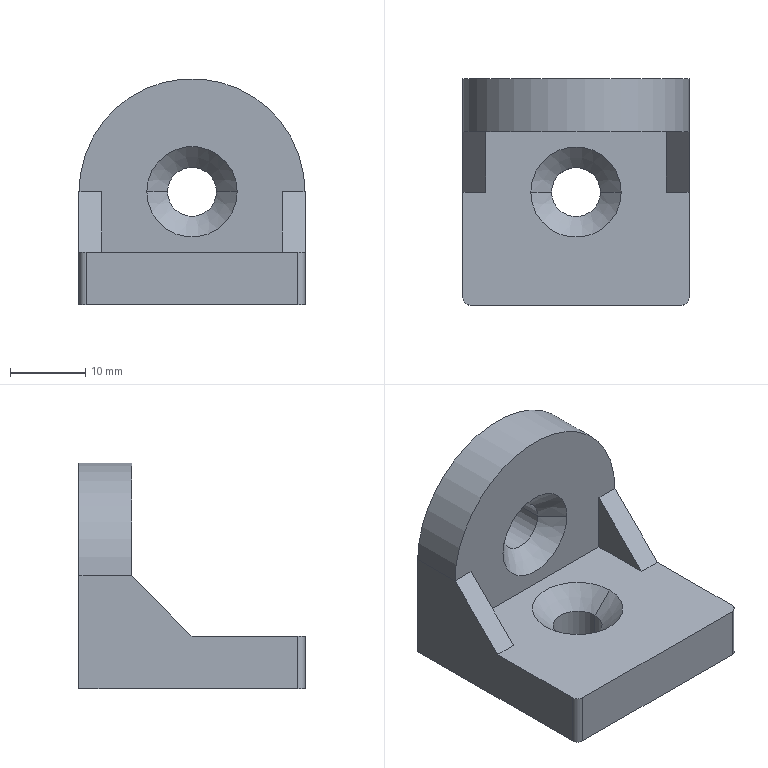Component | SolidWorks | TurningAnglePieceHDH[HDH-83030]_HDH-83030-1 | 1 solid | 22 faces | box 30 x 30 x 30 mm | volume 9980 mm3 | plane 11 | cylinder 7 | cone 4 | commonest cylinder face diameters 6.5 x4 2 x2 30 x1
STEP:
#1=COLOUR_RGB('',0.7922,0.8196,0.9333);
#2=FILL_AREA_STYLE_COLOUR('',#1);
#3=FILL_AREA_STYLE('',(#2));
#4=SURFACE_STYLE_FILL_AREA(#3);
#5=SURFACE_SIDE_STYLE('',(#4));
#6=SURFACE_STYLE_USAGE(.BOTH.,#5);
#7=PRESENTATION_STYLE_ASSIGNMENT((#6));
#8=CARTESIAN_POINT('',(-1.309,-1.969,0.315));
#9=VERTEX_POINT('',#8);
#10=CARTESIAN_POINT('',(-1.053,-1.969,0.315));
#11=VERTEX_POINT('',#10);
#12=CARTESIAN_POINT('',(-1.181,-1.969,0.315));
#13=DIRECTION('',(0.,0.,1.));
#14=DIRECTION('',(1.,0.,0.));
#15=AXIS2_PLACEMENT_3D('',#12,#13,#14);
#16=CIRCLE('',#15,0.128);
#17=EDGE_CURVE('',#9,#11,#16,.T.);
#18=ORIENTED_EDGE('',*,*,#17,.F.);
#19=CARTESIAN_POINT('',(-1.309,-1.969,0.4823));
#20=VERTEX_POINT('',#19);
#21=CARTESIAN_POINT('',(-1.309,-1.969,0.5906));
#22=DIRECTION('',(0.,0.,1.));
#23=VECTOR('',#22,39.37);
#24=LINE('',#21,#23);
#25=EDGE_CURVE('',#9,#20,#24,.T.);
#26=ORIENTED_EDGE('',*,*,#25,.T.);
#27=CARTESIAN_POINT('',(-1.053,-1.969,0.4823));
#28=VERTEX_POINT('',#27);
#29=CARTESIAN_POINT('',(-1.181,-1.969,0.4823));
#30=DIRECTION('',(0.,0.,-1.));
#31=DIRECTION('',(1.,0.,0.));
#32=AXIS2_PLACEMENT_3D('',#29,#30,#31);
#33=CIRCLE('',#32,0.128);
#34=EDGE_CURVE('',#28,#20,#33,.T.);
#35=ORIENTED_EDGE('',*,*,#34,.F.);
#36=CARTESIAN_POINT('',(-1.053,-1.969,0.5906));
#37=DIRECTION('',(0.,0.,1.));
#38=VECTOR('',#37,39.37);
#39=LINE('',#36,#38);
#40=EDGE_CURVE('',#11,#28,#39,.T.);
#41=ORIENTED_EDGE('',*,*,#40,.F.);
#42=EDGE_LOOP('',(#18,#26,#35,#41));
#43=FACE_OUTER_BOUND('',#42,.T.);
#44=CARTESIAN_POINT('',(-1.181,-1.969,0.5906));
#45=DIRECTION('',(0.,0.,1.));
#46=DIRECTION('',(1.,0.,0.));
#47=AXIS2_PLACEMENT_3D('',#44,#45,#46);
#48=CYLINDRICAL_SURFACE('',#47,0.128);
#49=ADVANCED_FACE('',(#43),#48,.F.);
#50=ORIENTED_EDGE('',*,*,#34,.T.);
#51=CARTESIAN_POINT('',(-1.417,-1.969,0.5906));
#52=VERTEX_POINT('',#51);
#53=CARTESIAN_POINT('',(-1.417,-1.969,0.5906));
#54=DIRECTION('',(-0.7071,0.,0.7071));
#55=VECTOR('',#54,39.37);
#56=LINE('',#53,#55);
#57=EDGE_CURVE('',#20,#52,#56,.T.);
#58=ORIENTED_EDGE('',*,*,#57,.T.);
#59=CARTESIAN_POINT('',(-0.9449,-1.969,0.5906));
#60=VERTEX_POINT('',#59);
#61=CARTESIAN_POINT('',(-1.181,-1.969,0.5906));
#62=DIRECTION('',(0.,0.,-1.));
#63=DIRECTION('',(1.,0.,0.));
#64=AXIS2_PLACEMENT_3D('',#61,#62,#63);
#65=CIRCLE('',#64,0.2362);
#66=EDGE_CURVE('',#60,#52,#65,.T.);
#67=ORIENTED_EDGE('',*,*,#66,.F.);
#68=CARTESIAN_POINT('',(-0.9449,-1.969,0.5906));
#69=DIRECTION('',(0.7071,0.,0.7071));
#70=VECTOR('',#69,39.37);
#71=LINE('',#68,#70);
#72=EDGE_CURVE('',#28,#60,#71,.T.);
#73=ORIENTED_EDGE('',*,*,#72,.F.);
#74=EDGE_LOOP('',(#50,#58,#67,#73));
#75=FACE_OUTER_BOUND('',#74,.T.);
#76=CARTESIAN_POINT('',(-1.181,-1.969,0.5906));
#77=DIRECTION('',(0.,0.,1.));
#78=DIRECTION('',(1.,0.,0.));
#79=AXIS2_PLACEMENT_3D('',#76,#77,#78);
#80=CONICAL_SURFACE('',#79,0.2362,0.7854);
#81=ADVANCED_FACE('',(#75),#80,.F.);
#82=CARTESIAN_POINT('',(-1.309,-1.378,0.9055));
#83=VERTEX_POINT('',#82);
#84=CARTESIAN_POINT('',(-1.053,-1.378,0.9055));
#85=VERTEX_POINT('',#84);
#86=CARTESIAN_POINT('',(-1.181,-1.378,0.9055));
#87=DIRECTION('',(0.,-1.,0.));
#88=DIRECTION('',(1.,0.,0.));
#89=AXIS2_PLACEMENT_3D('',#86,#87,#88);
#90=CIRCLE('',#89,0.128);
#91=EDGE_CURVE('',#83,#85,#90,.T.);
#92=ORIENTED_EDGE('',*,*,#91,.F.);
#93=CARTESIAN_POINT('',(-1.309,-1.545,0.9055));
#94=VERTEX_POINT('',#93);
#95=CARTESIAN_POINT('',(-1.309,-1.654,0.9055));
#96=DIRECTION('',(0.,-1.,0.));
#97=VECTOR('',#96,39.37);
#98=LINE('',#95,#97);
#99=EDGE_CURVE('',#83,#94,#98,.T.);
#100=ORIENTED_EDGE('',*,*,#99,.T.);
#101=CARTESIAN_POINT('',(-1.053,-1.545,0.9055));
#102=VERTEX_POINT('',#101);
#103=CARTESIAN_POINT('',(-1.181,-1.545,0.9055));
#104=DIRECTION('',(0.,1.,0.));
#105=DIRECTION('',(1.,0.,0.));
#106=AXIS2_PLACEMENT_3D('',#103,#104,#105);
#107=CIRCLE('',#106,0.128);
#108=EDGE_CURVE('',#102,#94,#107,.T.);
#109=ORIENTED_EDGE('',*,*,#108,.F.);
#110=CARTESIAN_POINT('',(-1.053,-1.654,0.9055));
#111=DIRECTION('',(0.,-1.,0.));
#112=VECTOR('',#111,39.37);
#113=LINE('',#110,#112);
#114=EDGE_CURVE('',#85,#102,#113,.T.);
#115=ORIENTED_EDGE('',*,*,#114,.F.);
#116=EDGE_LOOP('',(#92,#100,#109,#115));
#117=FACE_OUTER_BOUND('',#116,.T.);
#118=CARTESIAN_POINT('',(-1.181,-1.654,0.9055));
#119=DIRECTION('',(0.,-1.,0.));
#120=DIRECTION('',(1.,0.,0.));
#121=AXIS2_PLACEMENT_3D('',#118,#119,#120);
#122=CYLINDRICAL_SURFACE('',#121,0.128);
#123=ADVANCED_FACE('',(#117),#122,.F.);
#124=ORIENTED_EDGE('',*,*,#108,.T.);
#125=CARTESIAN_POINT('',(-1.417,-1.654,0.9055));
#126=VERTEX_POINT('',#125);
#127=CARTESIAN_POINT('',(-1.417,-1.654,0.9055));
#128=DIRECTION('',(-0.7071,-0.7071,0.));
#129=VECTOR('',#128,39.37);
#130=LINE('',#127,#129);
#131=EDGE_CURVE('',#94,#126,#130,.T.);
#132=ORIENTED_EDGE('',*,*,#131,.T.);
#133=CARTESIAN_POINT('',(-0.9449,-1.654,0.9055));
#134=VERTEX_POINT('',#133);
#135=CARTESIAN_POINT('',(-1.181,-1.654,0.9055));
#136=DIRECTION('',(0.,1.,0.));
#137=DIRECTION('',(1.,0.,0.));
#138=AXIS2_PLACEMENT_3D('',#135,#136,#137);
#139=CIRCLE('',#138,0.2362);
#140=EDGE_CURVE('',#134,#126,#139,.T.);
#141=ORIENTED_EDGE('',*,*,#140,.F.);
#142=CARTESIAN_POINT('',(-0.9449,-1.654,0.9055));
#143=DIRECTION('',(0.7071,-0.7071,0.));
#144=VECTOR('',#143,39.37);
#145=LINE('',#142,#144);
#146=EDGE_CURVE('',#102,#134,#145,.T.);
#147=ORIENTED_EDGE('',*,*,#146,.F.);
#148=EDGE_LOOP('',(#124,#132,#141,#147));
#149=FACE_OUTER_BOUND('',#148,.T.);
#150=CARTESIAN_POINT('',(-1.181,-1.654,0.9055));
#151=DIRECTION('',(0.,-1.,0.));
#152=DIRECTION('',(1.,0.,0.));
#153=AXIS2_PLACEMENT_3D('',#150,#151,#152);
#154=CONICAL_SURFACE('',#153,0.2362,0.7854);
#155=ADVANCED_FACE('',(#149),#154,.F.);
#156=CARTESIAN_POINT('',(-0.7087,-1.654,0.9055));
#157=VERTEX_POINT('',#156);
#158=CARTESIAN_POINT('',(-0.7087,-1.969,0.5906));
#159=VERTEX_POINT('',#158);
#160=CARTESIAN_POINT('',(-0.7087,-1.654,0.9055));
#161=DIRECTION('',(0.,-0.7071,-0.7071));
#162=VECTOR('',#161,39.37);
#163=LINE('',#160,#162);
#164=EDGE_CURVE('',#157,#159,#163,.T.);
#165=ORIENTED_EDGE('',*,*,#164,.F.);
#166=CARTESIAN_POINT('',(-0.7087,-1.654,0.5906));
#167=VERTEX_POINT('',#166);
#168=CARTESIAN_POINT('',(-0.7087,-1.654,1.496));
#169=DIRECTION('',(0.,0.,1.));
#170=VECTOR('',#169,39.37);
#171=LINE('',#168,#170);
#172=EDGE_CURVE('',#167,#157,#171,.T.);
#173=ORIENTED_EDGE('',*,*,#172,.F.);
#174=CARTESIAN_POINT('',(-0.7087,-1.654,0.5906));
#175=DIRECTION('',(0.,1.,0.));
#176=VECTOR('',#175,39.37);
#177=LINE('',#174,#176);
#178=EDGE_CURVE('',#159,#167,#177,.T.);
#179=ORIENTED_EDGE('',*,*,#178,.F.);
#180=EDGE_LOOP('',(#165,#173,#179));
#181=FACE_OUTER_BOUND('',#180,.T.);
#182=CARTESIAN_POINT('',(-0.7087,-1.378,0.315));
#183=DIRECTION('',(1.,0.,0.));
#184=DIRECTION('',(0.,1.,0.));
#185=AXIS2_PLACEMENT_3D('',#182,#183,#184);
#186=PLANE('',#185);
#187=ADVANCED_FACE('',(#181),#186,.F.);
#188=ORIENTED_EDGE('',*,*,#140,.T.);
#189=CARTESIAN_POINT('',(-1.181,-1.654,0.9055));
#190=DIRECTION('',(0.,1.,0.));
#191=DIRECTION('',(1.,0.,0.));
#192=AXIS2_PLACEMENT_3D('',#189,#190,#191);
#193=CIRCLE('',#192,0.2362);
#194=EDGE_CURVE('',#126,#134,#193,.T.);
#195=ORIENTED_EDGE('',*,*,#194,.T.);
#196=EDGE_LOOP('',(#188,#195));
#197=FACE_BOUND('',#196,.T.);
#198=CARTESIAN_POINT('',(-0.5906,-1.654,0.9055));
#199=VERTEX_POINT('',#198);
#200=CARTESIAN_POINT('',(-0.5906,-1.654,0.9055));
#201=DIRECTION('',(-1.,0.,0.));
#202=VECTOR('',#201,39.37);
#203=LINE('',#200,#202);
#204=EDGE_CURVE('',#199,#157,#203,.T.);
#205=ORIENTED_EDGE('',*,*,#204,.F.);
#206=CARTESIAN_POINT('',(-1.772,-1.654,0.9055));
#207=VERTEX_POINT('',#206);
#208=CARTESIAN_POINT('',(-1.181,-1.654,0.9055));
#209=DIRECTION('',(0.,1.,0.));
#210=DIRECTION('',(1.,0.,0.));
#211=AXIS2_PLACEMENT_3D('',#208,#209,#210);
#212=CIRCLE('',#211,0.5906);
#213=EDGE_CURVE('',#207,#199,#212,.T.);
#214=ORIENTED_EDGE('',*,*,#213,.F.);
#215=CARTESIAN_POINT('',(-1.654,-1.654,0.9055));
#216=VERTEX_POINT('',#215);
#217=CARTESIAN_POINT('',(-1.772,-1.654,0.9055));
#218=DIRECTION('',(1.,0.,0.));
#219=VECTOR('',#218,39.37);
#220=LINE('',#217,#219);
#221=EDGE_CURVE('',#207,#216,#220,.T.);
#222=ORIENTED_EDGE('',*,*,#221,.T.);
#223=CARTESIAN_POINT('',(-1.654,-1.654,0.5906));
#224=VERTEX_POINT('',#223);
#225=CARTESIAN_POINT('',(-1.654,-1.654,0.315));
#226=DIRECTION('',(0.,0.,1.));
#227=VECTOR('',#226,39.37);
#228=LINE('',#225,#227);
#229=EDGE_CURVE('',#224,#216,#228,.T.);
#230=ORIENTED_EDGE('',*,*,#229,.F.);
#231=CARTESIAN_POINT('',(-1.772,-1.654,0.5906));
#232=DIRECTION('',(-1.,0.,0.));
#233=VECTOR('',#232,39.37);
#234=LINE('',#231,#233);
#235=EDGE_CURVE('',#167,#224,#234,.T.);
#236=ORIENTED_EDGE('',*,*,#235,.F.);
#237=ORIENTED_EDGE('',*,*,#172,.T.);
#238=EDGE_LOOP('',(#205,#214,#222,#230,#236,#237));
#239=FACE_OUTER_BOUND('',#238,.T.);
#240=CARTESIAN_POINT('',(-1.772,-1.654,1.496));
#241=DIRECTION('',(0.,-1.,0.));
#242=DIRECTION('',(1.,0.,0.));
#243=AXIS2_PLACEMENT_3D('',#240,#241,#242);
#244=PLANE('',#243);
#245=ADVANCED_FACE('',(#197,#239),#244,.T.);
#246=ORIENTED_EDGE('',*,*,#229,.T.);
#247=CARTESIAN_POINT('',(-1.654,-1.969,0.5906));
#248=VERTEX_POINT('',#247);
#249=CARTESIAN_POINT('',(-1.654,-1.654,0.9055));
#250=DIRECTION('',(0.,-0.7071,-0.7071));
#251=VECTOR('',#250,39.37);
#252=LINE('',#249,#251);
#253=EDGE_CURVE('',#216,#248,#252,.T.);
#254=ORIENTED_EDGE('',*,*,#253,.T.);
#255=CARTESIAN_POINT('',(-1.654,-1.654,0.5906));
#256=DIRECTION('',(0.,-1.,0.));
#257=VECTOR('',#256,39.37);
#258=LINE('',#255,#257);
#259=EDGE_CURVE('',#224,#248,#258,.T.);
#260=ORIENTED_EDGE('',*,*,#259,.F.);
#261=EDGE_LOOP('',(#246,#254,#260));
#262=FACE_OUTER_BOUND('',#261,.T.);
#263=CARTESIAN_POINT('',(-1.654,-1.378,0.315));
#264=DIRECTION('',(1.,0.,0.));
#265=DIRECTION('',(0.,1.,0.));
#266=AXIS2_PLACEMENT_3D('',#263,#264,#265);
#267=PLANE('',#266);
#268=ADVANCED_FACE('',(#262),#267,.T.);
#269=CARTESIAN_POINT('',(-1.732,-2.559,0.5906));
#270=VERTEX_POINT('',#269);
#271=CARTESIAN_POINT('',(-1.732,-2.559,0.315));
#272=VERTEX_POINT('',#271);
#273=CARTESIAN_POINT('',(-1.732,-2.559,0.5906));
#274=DIRECTION('',(0.,0.,-1.));
#275=VECTOR('',#274,39.37);
#276=LINE('',#273,#275);
#277=EDGE_CURVE('',#270,#272,#276,.T.);
#278=ORIENTED_EDGE('',*,*,#277,.F.);
#279=CARTESIAN_POINT('',(-1.772,-2.52,0.5906));
#280=VERTEX_POINT('',#279);
#281=CARTESIAN_POINT('',(-1.732,-2.52,0.5906));
#282=DIRECTION('',(0.,0.,1.));
#283=DIRECTION('',(1.,0.,0.));
#284=AXIS2_PLACEMENT_3D('',#281,#282,#283);
#285=CIRCLE('',#284,0.03937);
#286=EDGE_CURVE('',#280,#270,#285,.T.);
#287=ORIENTED_EDGE('',*,*,#286,.F.);
#288=CARTESIAN_POINT('',(-1.772,-2.52,0.315));
#289=VERTEX_POINT('',#288);
#290=CARTESIAN_POINT('',(-1.772,-2.52,0.315));
#291=DIRECTION('',(0.,0.,-1.));
#292=VECTOR('',#291,39.37);
#293=LINE('',#290,#292);
#294=EDGE_CURVE('',#280,#289,#293,.T.);
#295=ORIENTED_EDGE('',*,*,#294,.T.);
#296=CARTESIAN_POINT('',(-1.732,-2.52,0.315));
#297=DIRECTION('',(0.,0.,1.));
#298=DIRECTION('',(1.,0.,0.));
#299=AXIS2_PLACEMENT_3D('',#296,#297,#298);
#300=CIRCLE('',#299,0.03937);
#301=EDGE_CURVE('',#289,#272,#300,.T.);
#302=ORIENTED_EDGE('',*,*,#301,.T.);
#303=EDGE_LOOP('',(#278,#287,#295,#302));
#304=FACE_OUTER_BOUND('',#303,.T.);
#305=CARTESIAN_POINT('',(-1.732,-2.52,-1.225));
#306=DIRECTION('',(0.,0.,1.));
#307=DIRECTION('',(1.,0.,0.));
#308=AXIS2_PLACEMENT_3D('',#305,#306,#307);
#309=CYLINDRICAL_SURFACE('',#308,0.03937);
#310=ADVANCED_FACE('',(#304),#309,.T.);
#311=ORIENTED_EDGE('',*,*,#253,.F.);
#312=ORIENTED_EDGE('',*,*,#221,.F.);
#313=CARTESIAN_POINT('',(-1.772,-1.969,0.5906));
#314=VERTEX_POINT('',#313);
#315=CARTESIAN_POINT('',(-1.772,-1.654,0.9055));
#316=DIRECTION('',(0.,-0.7071,-0.7071));
#317=VECTOR('',#316,39.37);
#318=LINE('',#315,#317);
#319=EDGE_CURVE('',#207,#314,#318,.T.);
#320=ORIENTED_EDGE('',*,*,#319,.T.);
#321=CARTESIAN_POINT('',(-1.772,-1.969,0.5906));
#322=DIRECTION('',(-1.,0.,0.));
#323=VECTOR('',#322,39.37);
#324=LINE('',#321,#323);
#325=EDGE_CURVE('',#248,#314,#324,.T.);
#326=ORIENTED_EDGE('',*,*,#325,.F.);
#327=EDGE_LOOP('',(#311,#312,#320,#326));
#328=FACE_OUTER_BOUND('',#327,.T.);
#329=CARTESIAN_POINT('',(-1.772,-1.654,0.9055));
#330=DIRECTION('',(0.,0.7071,-0.7071));
#331=DIRECTION('',(-1.,0.,0.));
#332=AXIS2_PLACEMENT_3D('',#329,#330,#331);
#333=PLANE('',#332);
#334=ADVANCED_FACE('',(#328),#333,.F.);
#335=CARTESIAN_POINT('',(-1.772,-1.378,0.9055));
#336=VERTEX_POINT('',#335);
#337=CARTESIAN_POINT('',(-1.772,-1.378,0.9055));
#338=DIRECTION('',(0.,-1.,0.));
#339=VECTOR('',#338,39.37);
#340=LINE('',#337,#339);
#341=EDGE_CURVE('',#336,#207,#340,.T.);
#342=ORIENTED_EDGE('',*,*,#341,.T.);
#343=ORIENTED_EDGE('',*,*,#213,.T.);
#344=CARTESIAN_POINT('',(-0.5906,-1.378,0.9055));
#345=VERTEX_POINT('',#344);
#346=CARTESIAN_POINT('',(-0.5906,-1.378,0.9055));
#347=DIRECTION('',(0.,-1.,0.));
#348=VECTOR('',#347,39.37);
#349=LINE('',#346,#348);
#350=EDGE_CURVE('',#345,#199,#349,.T.);
#351=ORIENTED_EDGE('',*,*,#350,.F.);
#352=CARTESIAN_POINT('',(-1.181,-1.378,0.9055));
#353=DIRECTION('',(0.,1.,0.));
#354=DIRECTION('',(1.,0.,0.));
#355=AXIS2_PLACEMENT_3D('',#352,#353,#354);
#356=CIRCLE('',#355,0.5906);
#357=EDGE_CURVE('',#336,#345,#356,.T.);
#358=ORIENTED_EDGE('',*,*,#357,.F.);
#359=EDGE_LOOP('',(#342,#343,#351,#358));
#360=FACE_OUTER_BOUND('',#359,.T.);
#361=CARTESIAN_POINT('',(-1.181,0.1617,0.9055));
#362=DIRECTION('',(0.,-1.,0.));
#363=DIRECTION('',(1.,0.,0.));
#364=AXIS2_PLACEMENT_3D('',#361,#362,#363);
#365=CYLINDRICAL_SURFACE('',#364,0.5906);
#366=ADVANCED_FACE('',(#360),#365,.T.);
#367=CARTESIAN_POINT('',(-0.5906,-1.969,0.5906));
#368=VERTEX_POINT('',#367);
#369=CARTESIAN_POINT('',(-0.5906,-1.654,0.9055));
#370=DIRECTION('',(0.,-0.7071,-0.7071));
#371=VECTOR('',#370,39.37);
#372=LINE('',#369,#371);
#373=EDGE_CURVE('',#199,#368,#372,.T.);
#374=ORIENTED_EDGE('',*,*,#373,.F.);
#375=ORIENTED_EDGE('',*,*,#204,.T.);
#376=ORIENTED_EDGE('',*,*,#164,.T.);
#377=CARTESIAN_POINT('',(-1.772,-1.969,0.5906));
#378=DIRECTION('',(-1.,0.,0.));
#379=VECTOR('',#378,39.37);
#380=LINE('',#377,#379);
#381=EDGE_CURVE('',#368,#159,#380,.T.);
#382=ORIENTED_EDGE('',*,*,#381,.F.);
#383=EDGE_LOOP('',(#374,#375,#376,#382));
#384=FACE_OUTER_BOUND('',#383,.T.);
#385=CARTESIAN_POINT('',(-0.5906,-1.654,0.9055));
#386=DIRECTION('',(0.,-0.7071,0.7071));
#387=DIRECTION('',(1.,0.,0.));
#388=AXIS2_PLACEMENT_3D('',#385,#386,#387);
#389=PLANE('',#388);
#390=ADVANCED_FACE('',(#384),#389,.T.);
#391=ORIENTED_EDGE('',*,*,#66,.T.);
#392=CARTESIAN_POINT('',(-1.181,-1.969,0.5906));
#393=DIRECTION('',(0.,0.,-1.));
#394=DIRECTION('',(1.,0.,0.));
#395=AXIS2_PLACEMENT_3D('',#392,#393,#394);
#396=CIRCLE('',#395,0.2362);
#397=EDGE_CURVE('',#52,#60,#396,.T.);
#398=ORIENTED_EDGE('',*,*,#397,.T.);
#399=EDGE_LOOP('',(#391,#398));
#400=FACE_BOUND('',#399,.T.);
#401=CARTESIAN_POINT('',(-0.6299,-2.559,0.5906));
#402=VERTEX_POINT('',#401);
#403=CARTESIAN_POINT('',(-1.772,-2.559,0.5906));
#404=DIRECTION('',(-1.,0.,0.));
#405=VECTOR('',#404,39.37);
#406=LINE('',#403,#405);
#407=EDGE_CURVE('',#402,#270,#406,.T.);
#408=ORIENTED_EDGE('',*,*,#407,.F.);
#409=CARTESIAN_POINT('',(-0.5906,-2.52,0.5906));
#410=VERTEX_POINT('',#409);
#411=CARTESIAN_POINT('',(-0.6299,-2.52,0.5906));
#412=DIRECTION('',(0.,0.,-1.));
#413=DIRECTION('',(-1.,0.,0.));
#414=AXIS2_PLACEMENT_3D('',#411,#412,#413);
#415=CIRCLE('',#414,0.03937);
#416=EDGE_CURVE('',#410,#402,#415,.T.);
#417=ORIENTED_EDGE('',*,*,#416,.F.);
#418=CARTESIAN_POINT('',(-0.5906,-1.378,0.5906));
#419=DIRECTION('',(0.,-1.,0.));
#420=VECTOR('',#419,39.37);
#421=LINE('',#418,#420);
#422=EDGE_CURVE('',#368,#410,#421,.T.);
#423=ORIENTED_EDGE('',*,*,#422,.F.);
#424=ORIENTED_EDGE('',*,*,#381,.T.);
#425=ORIENTED_EDGE('',*,*,#178,.T.);
#426=ORIENTED_EDGE('',*,*,#235,.T.);
#427=ORIENTED_EDGE('',*,*,#259,.T.);
#428=ORIENTED_EDGE('',*,*,#325,.T.);
#429=CARTESIAN_POINT('',(-1.772,-1.378,0.5906));
#430=DIRECTION('',(0.,-1.,0.));
#431=VECTOR('',#430,39.37);
#432=LINE('',#429,#431);
#433=EDGE_CURVE('',#314,#280,#432,.T.);
#434=ORIENTED_EDGE('',*,*,#433,.T.);
#435=ORIENTED_EDGE('',*,*,#286,.T.);
#436=EDGE_LOOP('',(#408,#417,#423,#424,#425,#426,#427,#428,#434,#435));
#437=FACE_OUTER_BOUND('',#436,.T.);
#438=CARTESIAN_POINT('',(-1.772,-1.654,0.5906));
#439=DIRECTION('',(0.,0.,1.));
#440=DIRECTION('',(0.,1.,0.));
#441=AXIS2_PLACEMENT_3D('',#438,#439,#440);
#442=PLANE('',#441);
#443=ADVANCED_FACE('',(#400,#437),#442,.T.);
#444=CARTESIAN_POINT('',(-0.6299,-2.559,0.315));
#445=VERTEX_POINT('',#444);
#446=CARTESIAN_POINT('',(-0.6299,-2.559,0.5906));
#447=DIRECTION('',(0.,0.,1.));
#448=VECTOR('',#447,39.37);
#449=LINE('',#446,#448);
#450=EDGE_CURVE('',#445,#402,#449,.T.);
#451=ORIENTED_EDGE('',*,*,#450,.F.);
#452=CARTESIAN_POINT('',(-0.5906,-2.52,0.315));
#453=VERTEX_POINT('',#452);
#454=CARTESIAN_POINT('',(-0.6299,-2.52,0.315));
#455=DIRECTION('',(0.,0.,1.));
#456=DIRECTION('',(-1.,0.,0.));
#457=AXIS2_PLACEMENT_3D('',#454,#455,#456);
#458=CIRCLE('',#457,0.03937);
#459=EDGE_CURVE('',#445,#453,#458,.T.);
#460=ORIENTED_EDGE('',*,*,#459,.T.);
#461=CARTESIAN_POINT('',(-0.5906,-2.52,0.315));
#462=DIRECTION('',(0.,0.,-1.));
#463=VECTOR('',#462,39.37);
#464=LINE('',#461,#463);
#465=EDGE_CURVE('',#410,#453,#464,.T.);
#466=ORIENTED_EDGE('',*,*,#465,.F.);
#467=ORIENTED_EDGE('',*,*,#416,.T.);
#468=EDGE_LOOP('',(#451,#460,#466,#467));
#469=FACE_OUTER_BOUND('',#468,.T.);
#470=CARTESIAN_POINT('',(-0.6299,-2.52,3.036));
#471=DIRECTION('',(0.,0.,-1.));
#472=DIRECTION('',(-1.,0.,0.));
#473=AXIS2_PLACEMENT_3D('',#470,#471,#472);
#474=CYLINDRICAL_SURFACE('',#473,0.03937);
#475=ADVANCED_FACE('',(#469),#474,.T.);
#476=CARTESIAN_POINT('',(-1.772,-2.559,0.315));
#477=DIRECTION('',(-1.,0.,0.));
#478=VECTOR('',#477,39.37);
#479=LINE('',#476,#478);
#480=EDGE_CURVE('',#445,#272,#479,.T.);
#481=ORIENTED_EDGE('',*,*,#480,.F.);
#482=ORIENTED_EDGE('',*,*,#450,.T.);
#483=ORIENTED_EDGE('',*,*,#407,.T.);
#484=ORIENTED_EDGE('',*,*,#277,.T.);
#485=EDGE_LOOP('',(#481,#482,#483,#484));
#486=FACE_OUTER_BOUND('',#485,.T.);
#487=CARTESIAN_POINT('',(-1.772,-2.559,0.5906));
#488=DIRECTION('',(0.,-1.,0.));
#489=DIRECTION('',(1.,0.,0.));
#490=AXIS2_PLACEMENT_3D('',#487,#488,#489);
#491=PLANE('',#490);
#492=ADVANCED_FACE('',(#486),#491,.T.);
#493=ORIENTED_EDGE('',*,*,#319,.F.);
#494=ORIENTED_EDGE('',*,*,#341,.F.);
#495=CARTESIAN_POINT('',(-1.772,-1.378,0.315));
#496=VERTEX_POINT('',#495);
#497=CARTESIAN_POINT('',(-1.772,-1.378,0.315));
#498=DIRECTION('',(0.,0.,1.));
#499=VECTOR('',#498,39.37);
#500=LINE('',#497,#499);
#501=EDGE_CURVE('',#496,#336,#500,.T.);
#502=ORIENTED_EDGE('',*,*,#501,.F.);
#503=CARTESIAN_POINT('',(-1.772,-2.559,0.315));
#504=DIRECTION('',(0.,1.,0.));
#505=VECTOR('',#504,39.37);
#506=LINE('',#503,#505);
#507=EDGE_CURVE('',#289,#496,#506,.T.);
#508=ORIENTED_EDGE('',*,*,#507,.F.);
#509=ORIENTED_EDGE('',*,*,#294,.F.);
#510=ORIENTED_EDGE('',*,*,#433,.F.);
#511=EDGE_LOOP('',(#493,#494,#502,#508,#509,#510));
#512=FACE_OUTER_BOUND('',#511,.T.);
#513=CARTESIAN_POINT('',(-1.772,-1.378,0.315));
#514=DIRECTION('',(1.,0.,0.));
#515=DIRECTION('',(0.,1.,0.));
#516=AXIS2_PLACEMENT_3D('',#513,#514,#515);
#517=PLANE('',#516);
#518=ADVANCED_FACE('',(#512),#517,.F.);
#519=CARTESIAN_POINT('',(-1.181,-1.378,0.9055));
#520=DIRECTION('',(0.,-1.,0.));
#521=DIRECTION('',(1.,0.,0.));
#522=AXIS2_PLACEMENT_3D('',#519,#520,#521);
#523=CIRCLE('',#522,0.128);
#524=EDGE_CURVE('',#85,#83,#523,.T.);
#525=ORIENTED_EDGE('',*,*,#524,.T.);
#526=ORIENTED_EDGE('',*,*,#91,.T.);
#527=EDGE_LOOP('',(#525,#526));
#528=FACE_BOUND('',#527,.T.);
#529=ORIENTED_EDGE('',*,*,#501,.T.);
#530=ORIENTED_EDGE('',*,*,#357,.T.);
#531=CARTESIAN_POINT('',(-0.5906,-1.378,0.315));
#532=VERTEX_POINT('',#531);
#533=CARTESIAN_POINT('',(-0.5906,-1.378,0.315));
#534=DIRECTION('',(0.,0.,1.));
#535=VECTOR('',#534,39.37);
#536=LINE('',#533,#535);
#537=EDGE_CURVE('',#532,#345,#536,.T.);
#538=ORIENTED_EDGE('',*,*,#537,.F.);
#539=CARTESIAN_POINT('',(-1.772,-1.378,0.315));
#540=DIRECTION('',(1.,0.,0.));
#541=VECTOR('',#540,39.37);
#542=LINE('',#539,#541);
#543=EDGE_CURVE('',#496,#532,#542,.T.);
#544=ORIENTED_EDGE('',*,*,#543,.F.);
#545=EDGE_LOOP('',(#529,#530,#538,#544));
#546=FACE_OUTER_BOUND('',#545,.T.);
#547=CARTESIAN_POINT('',(-1.772,-1.378,0.315));
#548=DIRECTION('',(0.,1.,0.));
#549=DIRECTION('',(0.,0.,1.));
#550=AXIS2_PLACEMENT_3D('',#547,#548,#549);
#551=PLANE('',#550);
#552=ADVANCED_FACE('',(#528,#546),#551,.T.);
#553=ORIENTED_EDGE('',*,*,#422,.T.);
#554=ORIENTED_EDGE('',*,*,#465,.T.);
#555=CARTESIAN_POINT('',(-0.5906,-2.559,0.315));
#556=DIRECTION('',(0.,-1.,0.));
#557=VECTOR('',#556,39.37);
#558=LINE('',#555,#557);
#559=EDGE_CURVE('',#532,#453,#558,.T.);
#560=ORIENTED_EDGE('',*,*,#559,.F.);
#561=ORIENTED_EDGE('',*,*,#537,.T.);
#562=ORIENTED_EDGE('',*,*,#350,.T.);
#563=ORIENTED_EDGE('',*,*,#373,.T.);
#564=EDGE_LOOP('',(#553,#554,#560,#561,#562,#563));
#565=FACE_OUTER_BOUND('',#564,.T.);
#566=CARTESIAN_POINT('',(-0.5906,-1.378,0.315));
#567=DIRECTION('',(1.,0.,0.));
#568=DIRECTION('',(0.,1.,0.));
#569=AXIS2_PLACEMENT_3D('',#566,#567,#568);
#570=PLANE('',#569);
#571=ADVANCED_FACE('',(#565),#570,.T.);
#572=CARTESIAN_POINT('',(-1.181,-1.969,0.315));
#573=DIRECTION('',(0.,0.,1.));
#574=DIRECTION('',(1.,0.,0.));
#575=AXIS2_PLACEMENT_3D('',#572,#573,#574);
#576=CIRCLE('',#575,0.128);
#577=EDGE_CURVE('',#11,#9,#576,.T.);
#578=ORIENTED_EDGE('',*,*,#577,.T.);
#579=ORIENTED_EDGE('',*,*,#17,.T.);
#580=EDGE_LOOP('',(#578,#579));
#581=FACE_BOUND('',#580,.T.);
#582=ORIENTED_EDGE('',*,*,#559,.T.);
#583=ORIENTED_EDGE('',*,*,#459,.F.);
#584=ORIENTED_EDGE('',*,*,#480,.T.);
#585=ORIENTED_EDGE('',*,*,#301,.F.);
#586=ORIENTED_EDGE('',*,*,#507,.T.);
#587=ORIENTED_EDGE('',*,*,#543,.T.);
#588=EDGE_LOOP('',(#582,#583,#584,#585,#586,#587));
#589=FACE_OUTER_BOUND('',#588,.T.);
#590=CARTESIAN_POINT('',(-1.772,-2.559,0.315));
#591=DIRECTION('',(0.,0.,-1.));
#592=DIRECTION('',(-1.,0.,0.));
#593=AXIS2_PLACEMENT_3D('',#590,#591,#592);
#594=PLANE('',#593);
#595=ADVANCED_FACE('',(#581,#589),#594,.T.);
#596=ORIENTED_EDGE('',*,*,#131,.F.);
#597=CARTESIAN_POINT('',(-1.181,-1.545,0.9055));
#598=DIRECTION('',(0.,1.,0.));
#599=DIRECTION('',(1.,0.,0.));
#600=AXIS2_PLACEMENT_3D('',#597,#598,#599);
#601=CIRCLE('',#600,0.128);
#602=EDGE_CURVE('',#94,#102,#601,.T.);
#603=ORIENTED_EDGE('',*,*,#602,.T.);
#604=ORIENTED_EDGE('',*,*,#146,.T.);
#605=ORIENTED_EDGE('',*,*,#194,.F.);
#606=EDGE_LOOP('',(#596,#603,#604,#605));
#607=FACE_OUTER_BOUND('',#606,.T.);
#608=CARTESIAN_POINT('',(-1.181,-1.654,0.9055));
#609=DIRECTION('',(0.,-1.,0.));
#610=DIRECTION('',(1.,0.,0.));
#611=AXIS2_PLACEMENT_3D('',#608,#609,#610);
#612=CONICAL_SURFACE('',#611,0.2362,0.7854);
#613=ADVANCED_FACE('',(#607),#612,.F.);
#614=ORIENTED_EDGE('',*,*,#99,.F.);
#615=ORIENTED_EDGE('',*,*,#524,.F.);
#616=ORIENTED_EDGE('',*,*,#114,.T.);
#617=ORIENTED_EDGE('',*,*,#602,.F.);
#618=EDGE_LOOP('',(#614,#615,#616,#617));
#619=FACE_OUTER_BOUND('',#618,.T.);
#620=CARTESIAN_POINT('',(-1.181,-1.654,0.9055));
#621=DIRECTION('',(0.,-1.,0.));
#622=DIRECTION('',(1.,0.,0.));
#623=AXIS2_PLACEMENT_3D('',#620,#621,#622);
#624=CYLINDRICAL_SURFACE('',#623,0.128);
#625=ADVANCED_FACE('',(#619),#624,.F.);
#626=ORIENTED_EDGE('',*,*,#57,.F.);
#627=CARTESIAN_POINT('',(-1.181,-1.969,0.4823));
#628=DIRECTION('',(0.,0.,-1.));
#629=DIRECTION('',(1.,0.,0.));
#630=AXIS2_PLACEMENT_3D('',#627,#628,#629);
#631=CIRCLE('',#630,0.128);
#632=EDGE_CURVE('',#20,#28,#631,.T.);
#633=ORIENTED_EDGE('',*,*,#632,.T.);
#634=ORIENTED_EDGE('',*,*,#72,.T.);
#635=ORIENTED_EDGE('',*,*,#397,.F.);
#636=EDGE_LOOP('',(#626,#633,#634,#635));
#637=FACE_OUTER_BOUND('',#636,.T.);
#638=CARTESIAN_POINT('',(-1.181,-1.969,0.5906));
#639=DIRECTION('',(0.,0.,1.));
#640=DIRECTION('',(1.,0.,0.));
#641=AXIS2_PLACEMENT_3D('',#638,#639,#640);
#642=CONICAL_SURFACE('',#641,0.2362,0.7854);
#643=ADVANCED_FACE('',(#637),#642,.F.);
#644=ORIENTED_EDGE('',*,*,#25,.F.);
#645=ORIENTED_EDGE('',*,*,#577,.F.);
#646=ORIENTED_EDGE('',*,*,#40,.T.);
#647=ORIENTED_EDGE('',*,*,#632,.F.);
#648=EDGE_LOOP('',(#644,#645,#646,#647));
#649=FACE_OUTER_BOUND('',#648,.T.);
#650=CARTESIAN_POINT('',(-1.181,-1.969,0.5906));
#651=DIRECTION('',(0.,0.,1.));
#652=DIRECTION('',(1.,0.,0.));
#653=AXIS2_PLACEMENT_3D('',#650,#651,#652);
#654=CYLINDRICAL_SURFACE('',#653,0.128);
#655=ADVANCED_FACE('',(#649),#654,.F.);
#656=CLOSED_SHELL('',(#49,#81,#123,#155,#187,#245,#268,#310,#334,#366,#390,#443,#475,#492,#518,#552,#571,#595,#613,#625,#643,#655));
#657=MANIFOLD_SOLID_BREP('',#656);
#658=STYLED_ITEM('',(#7),#657);
#659=PRESENTATION_LAYER_ASSIGNMENT('','',(#658));
#660=(LENGTH_UNIT()NAMED_UNIT(*)SI_UNIT($,.METRE.));
#661=LENGTH_MEASURE_WITH_UNIT(LENGTH_MEASURE(0.0254),#660);
#662=DIMENSIONAL_EXPONENTS(1.,0.,0.,0.,0.,0.,0.);
#663=(CONVERSION_BASED_UNIT('',#661)LENGTH_UNIT()NAMED_UNIT(#662));
#664=UNCERTAINTY_MEASURE_WITH_UNIT(LENGTH_MEASURE(0.00001),#663,'','');
#665=(NAMED_UNIT(*)PLANE_ANGLE_UNIT()SI_UNIT($,.RADIAN.));
#666=(NAMED_UNIT(*)SI_UNIT($,.STERADIAN.)SOLID_ANGLE_UNIT());
#667=(GEOMETRIC_REPRESENTATION_CONTEXT(3)GLOBAL_UNCERTAINTY_ASSIGNED_CONTEXT((#664))GLOBAL_UNIT_ASSIGNED_CONTEXT((#663,#665,#666))REPRESENTATION_CONTEXT('',''));
#668=MECHANICAL_DESIGN_GEOMETRIC_PRESENTATION_REPRESENTATION('',(#658),#667);
#669=CARTESIAN_POINT('',(0.,0.,0.));
#670=DIRECTION('',(0.,0.,1.));
#671=DIRECTION('',(1.,0.,0.));
#672=AXIS2_PLACEMENT_3D('',#669,#670,#671);
#673=(LENGTH_UNIT()NAMED_UNIT(*)SI_UNIT($,.METRE.));
#674=LENGTH_MEASURE_WITH_UNIT(LENGTH_MEASURE(0.0254),#673);
#675=DIMENSIONAL_EXPONENTS(1.,0.,0.,0.,0.,0.,0.);
#676=(CONVERSION_BASED_UNIT('',#674)LENGTH_UNIT()NAMED_UNIT(#675));
#677=UNCERTAINTY_MEASURE_WITH_UNIT(LENGTH_MEASURE(0.00001),#676,'','');
#678=(NAMED_UNIT(*)PLANE_ANGLE_UNIT()SI_UNIT($,.RADIAN.));
#679=(NAMED_UNIT(*)SI_UNIT($,.STERADIAN.)SOLID_ANGLE_UNIT());
#680=(GEOMETRIC_REPRESENTATION_CONTEXT(3)GLOBAL_UNCERTAINTY_ASSIGNED_CONTEXT((#677))GLOBAL_UNIT_ASSIGNED_CONTEXT((#676,#678,#679))REPRESENTATION_CONTEXT('',''));
#681=ADVANCED_BREP_SHAPE_REPRESENTATION('',(#657,#672),#680);